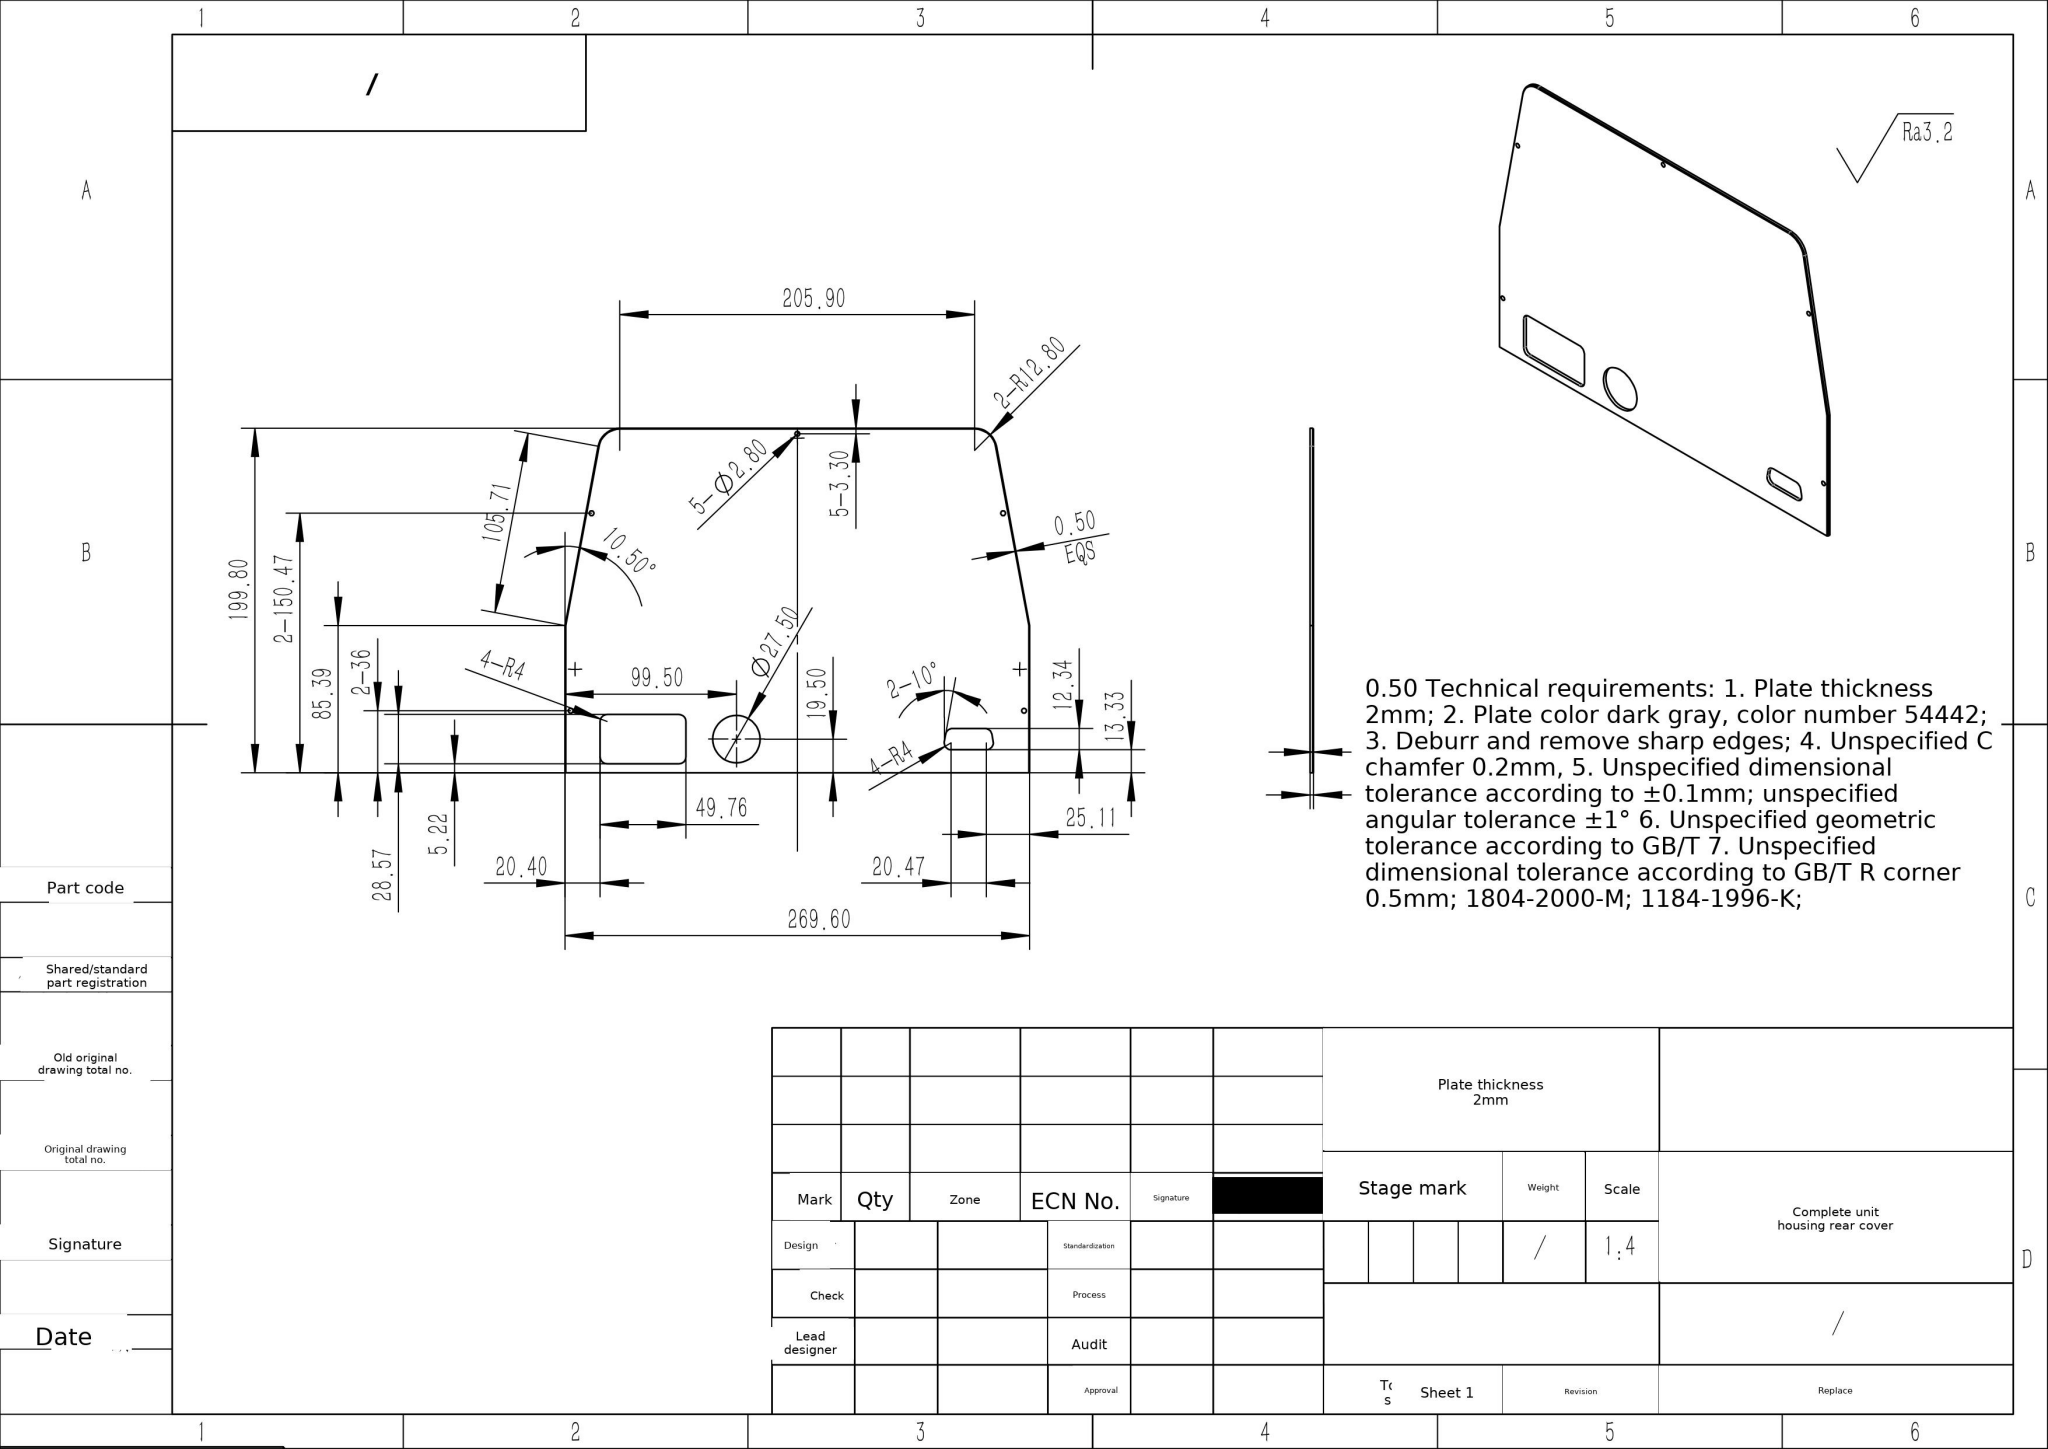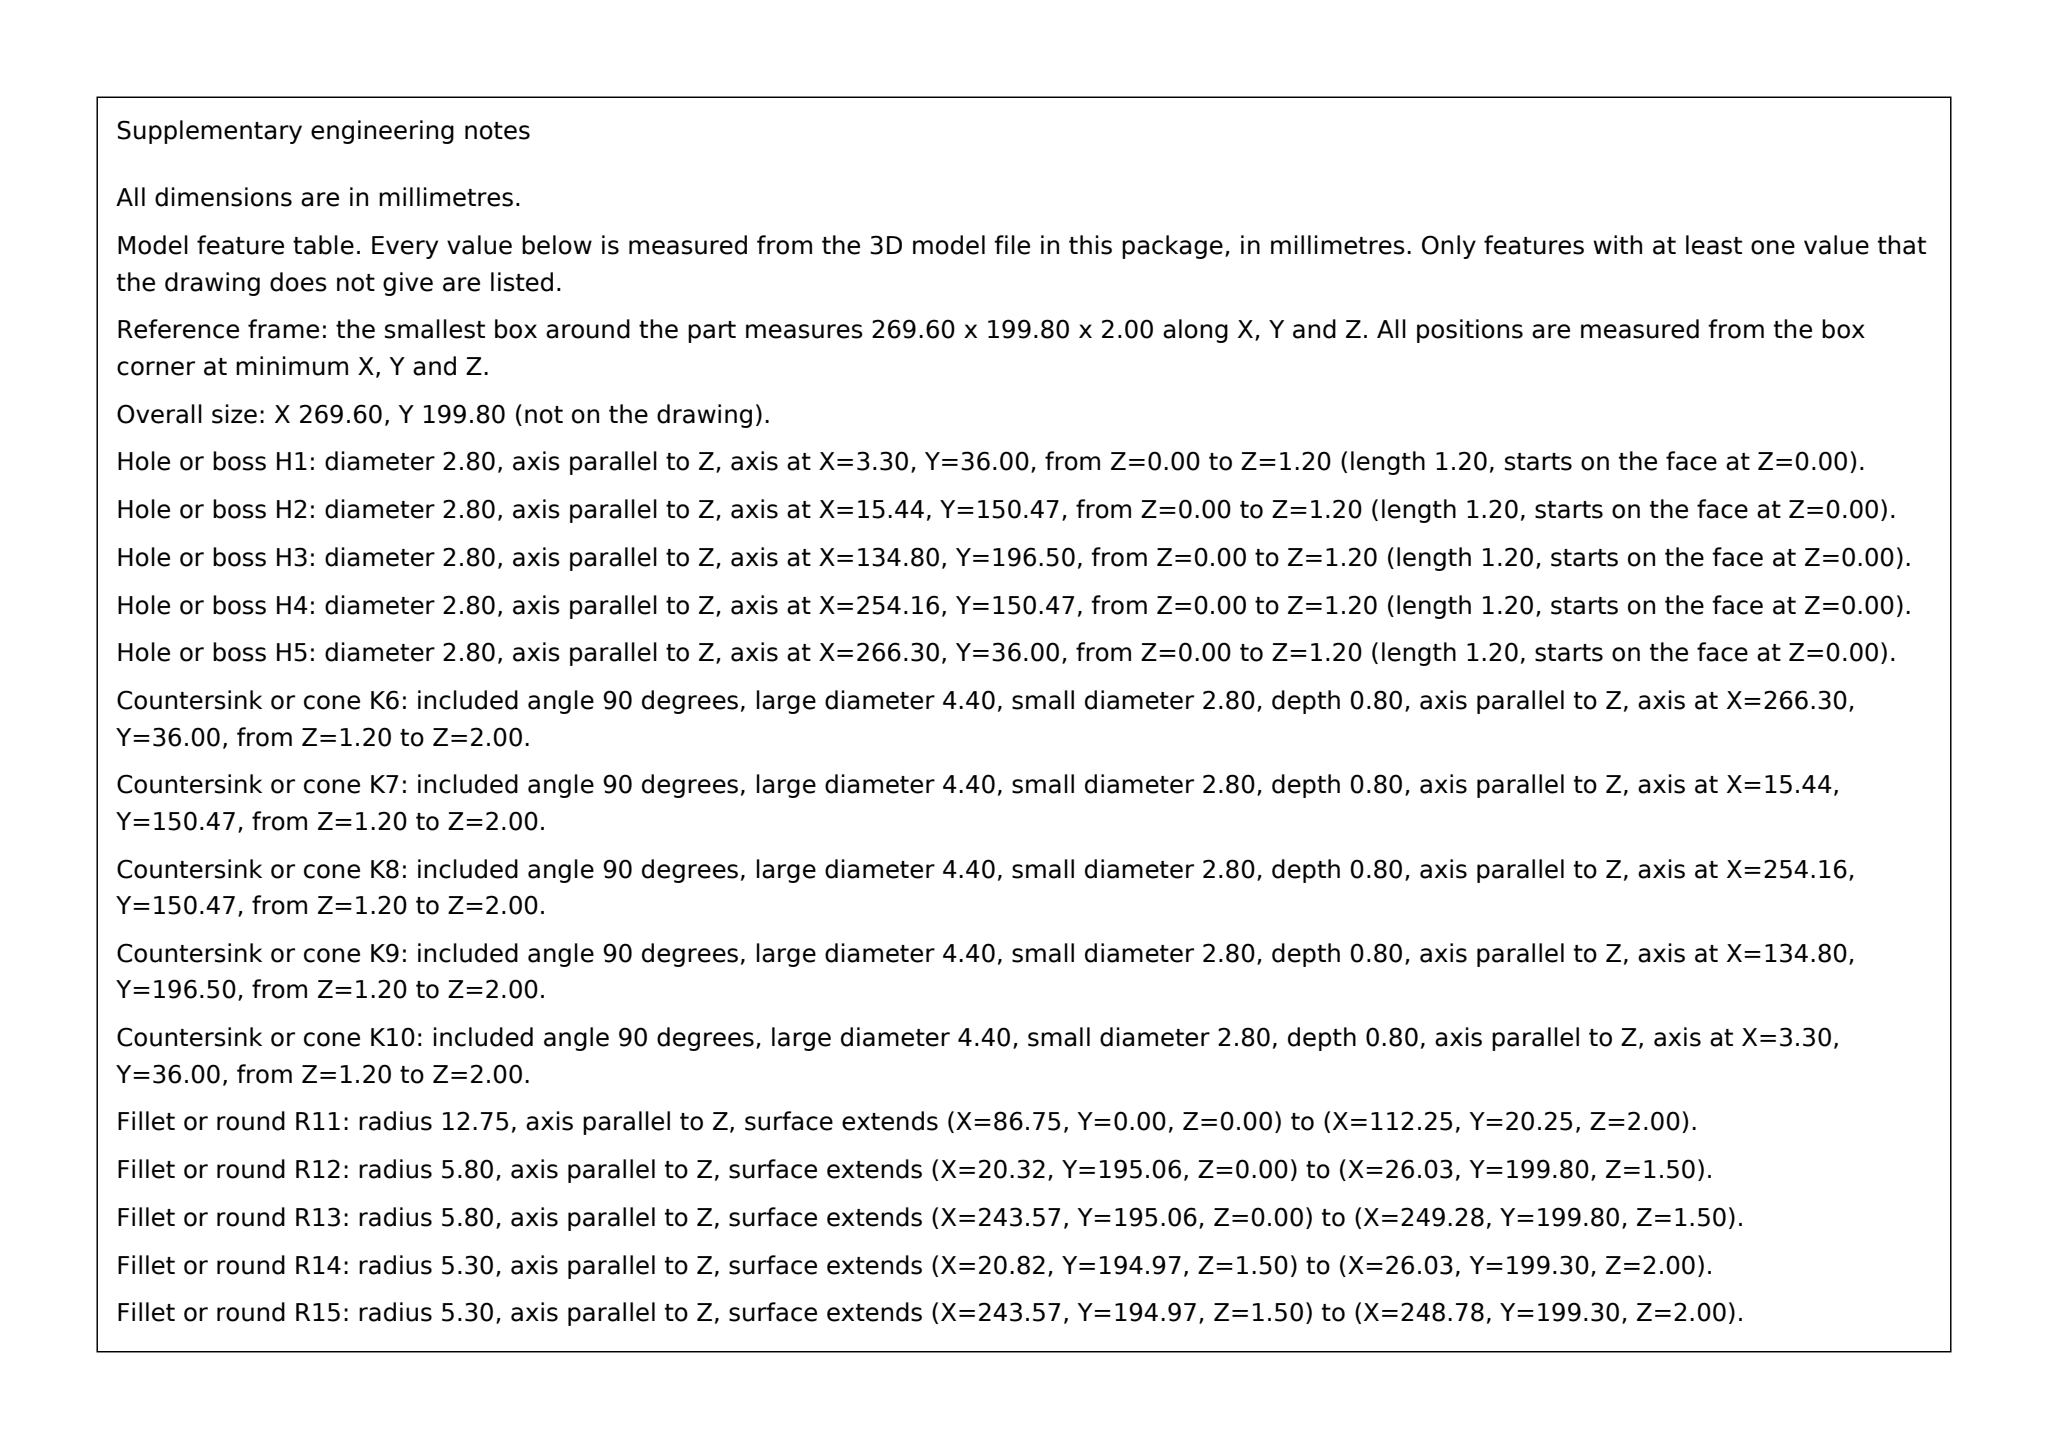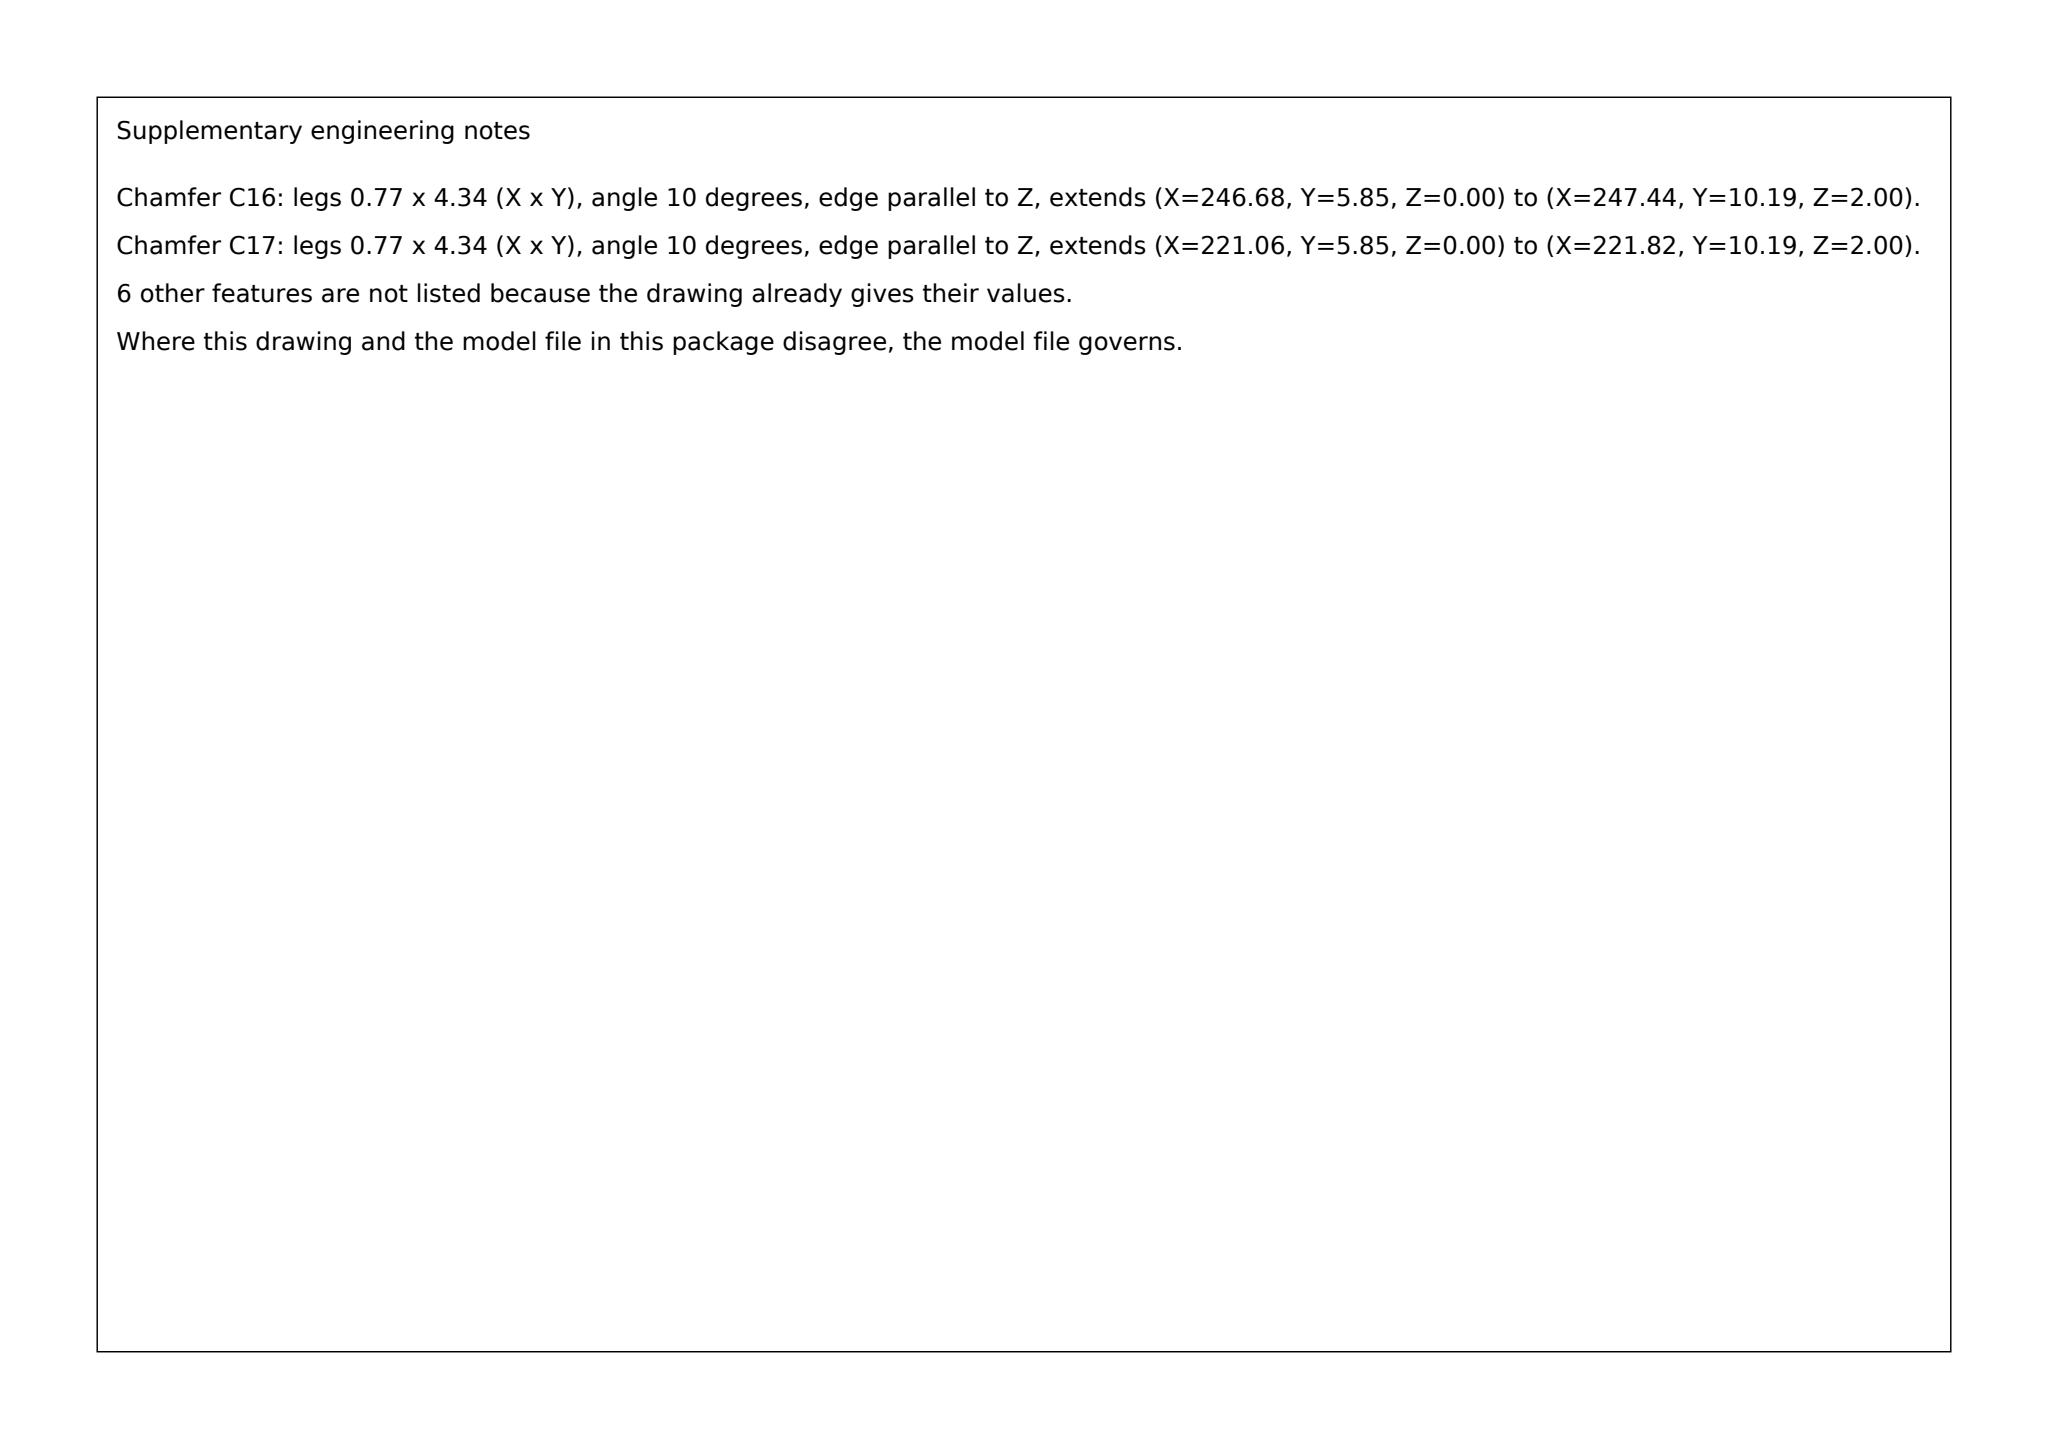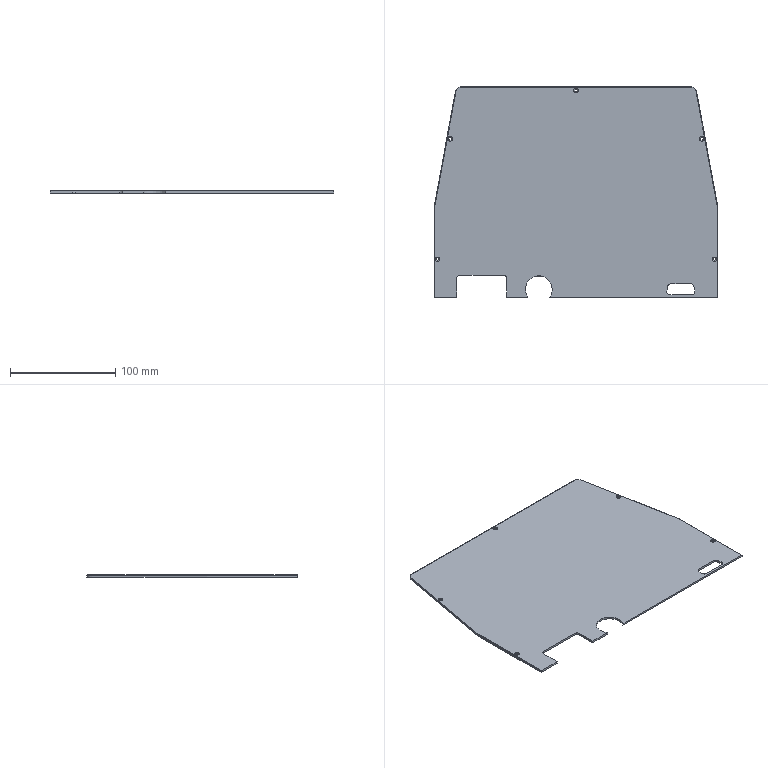Part | SolidWorks | mm | 1 solid | 57 faces | box 269.6 x 199.8 x 2 mm | volume 99263 mm3 | cylinder 24 | plane 23 | cone 10 | commonest cylinder face diameters 2.8 x10 6 x7 25.5 x3 10.6 x2 11.6 x2